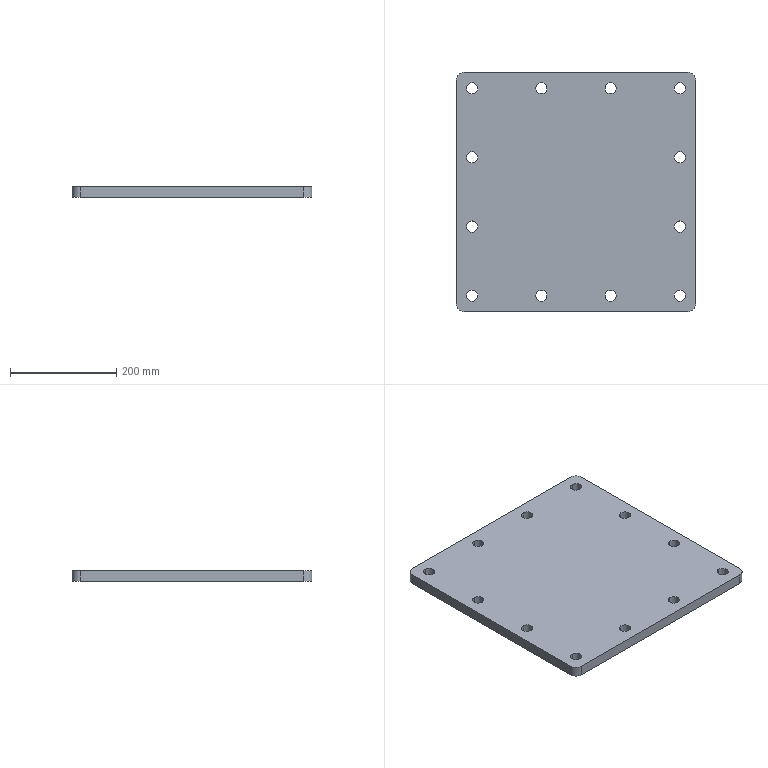Component | SolidWorks | TrolleyLeg-1_450X450X20-4 | 1 solid | 34 faces | volume 3963011 mm3 | cylinder 28 | plane 6 | commonest cylinder face diameters 21 x24 30 x4 | material Plain Carbon Steel